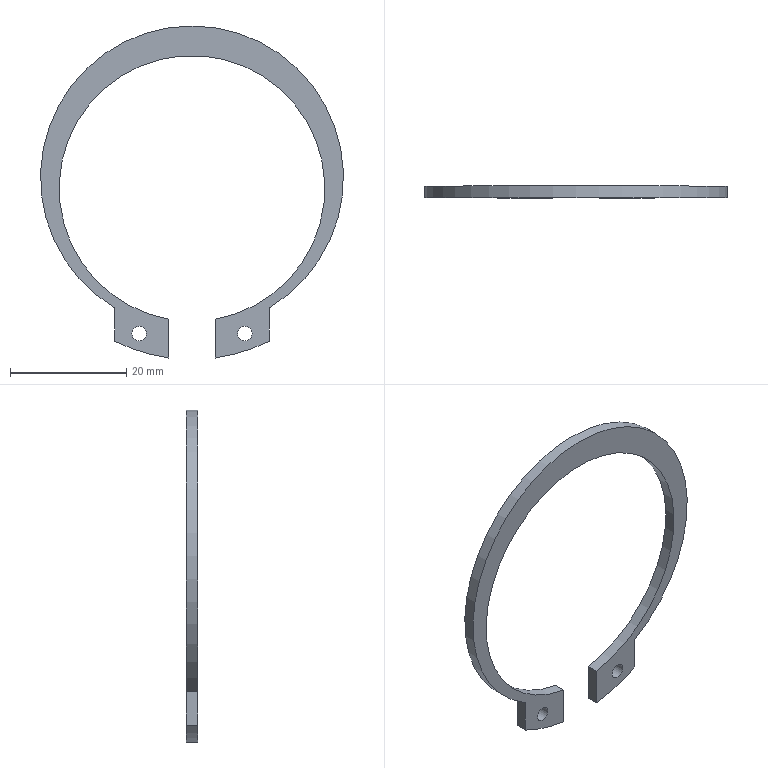Component | NX | SNAP_RING_2 | 1 solid | 12 faces | volume 1155 mm3 | plane 6 | cylinder 6 | commonest cylinder face diameters 59.014 x2 2.5 x2 45.8 x1 52.235 x1